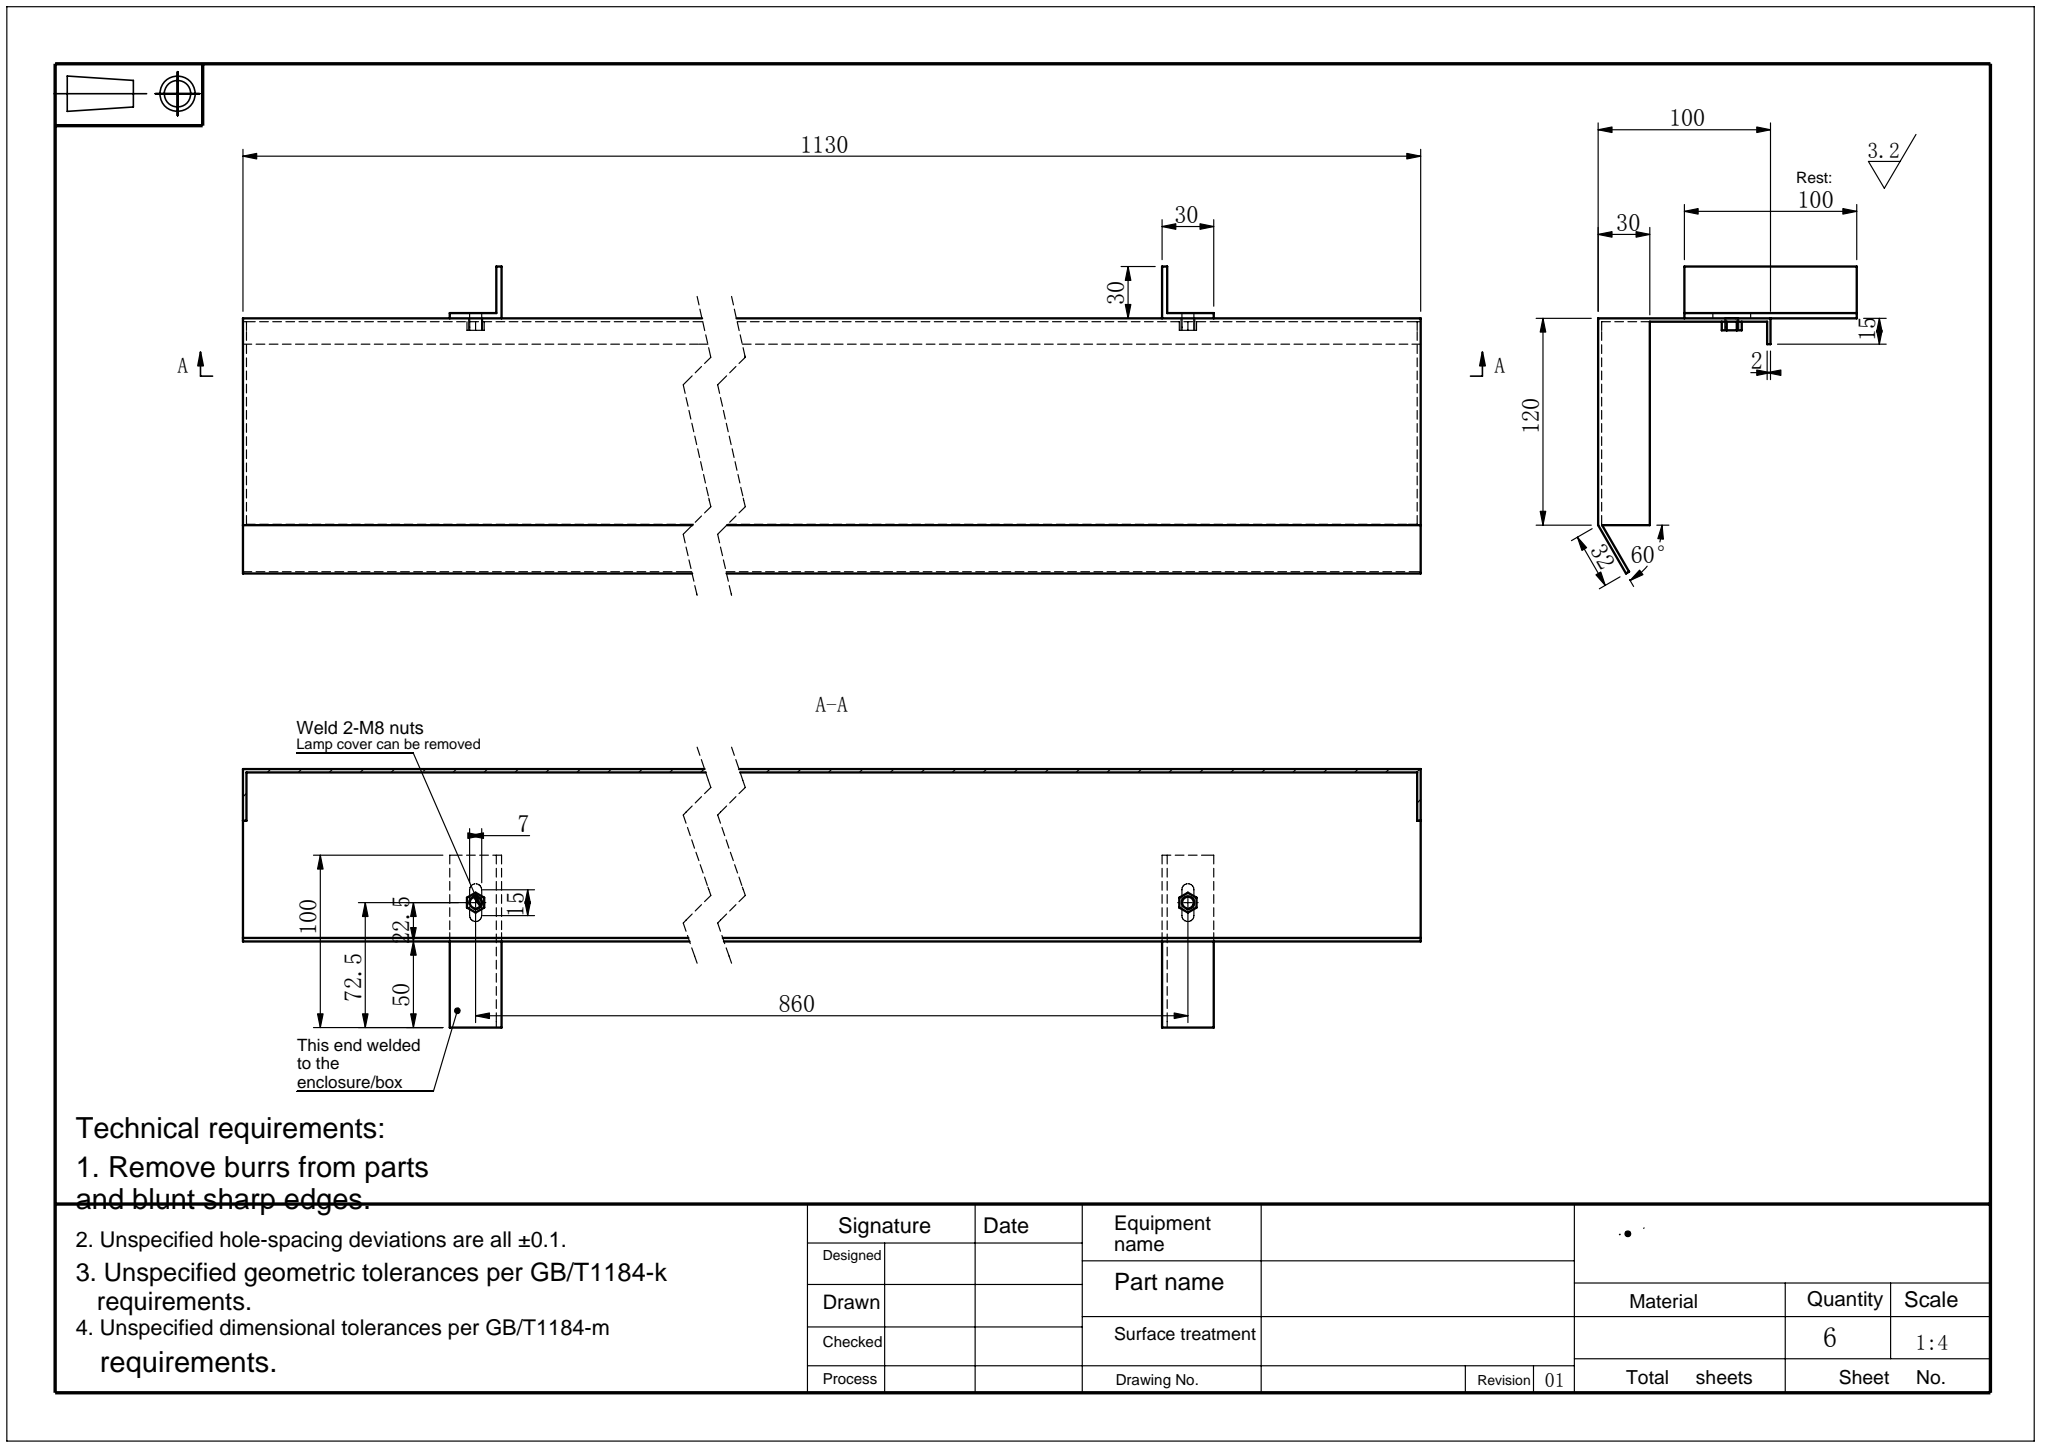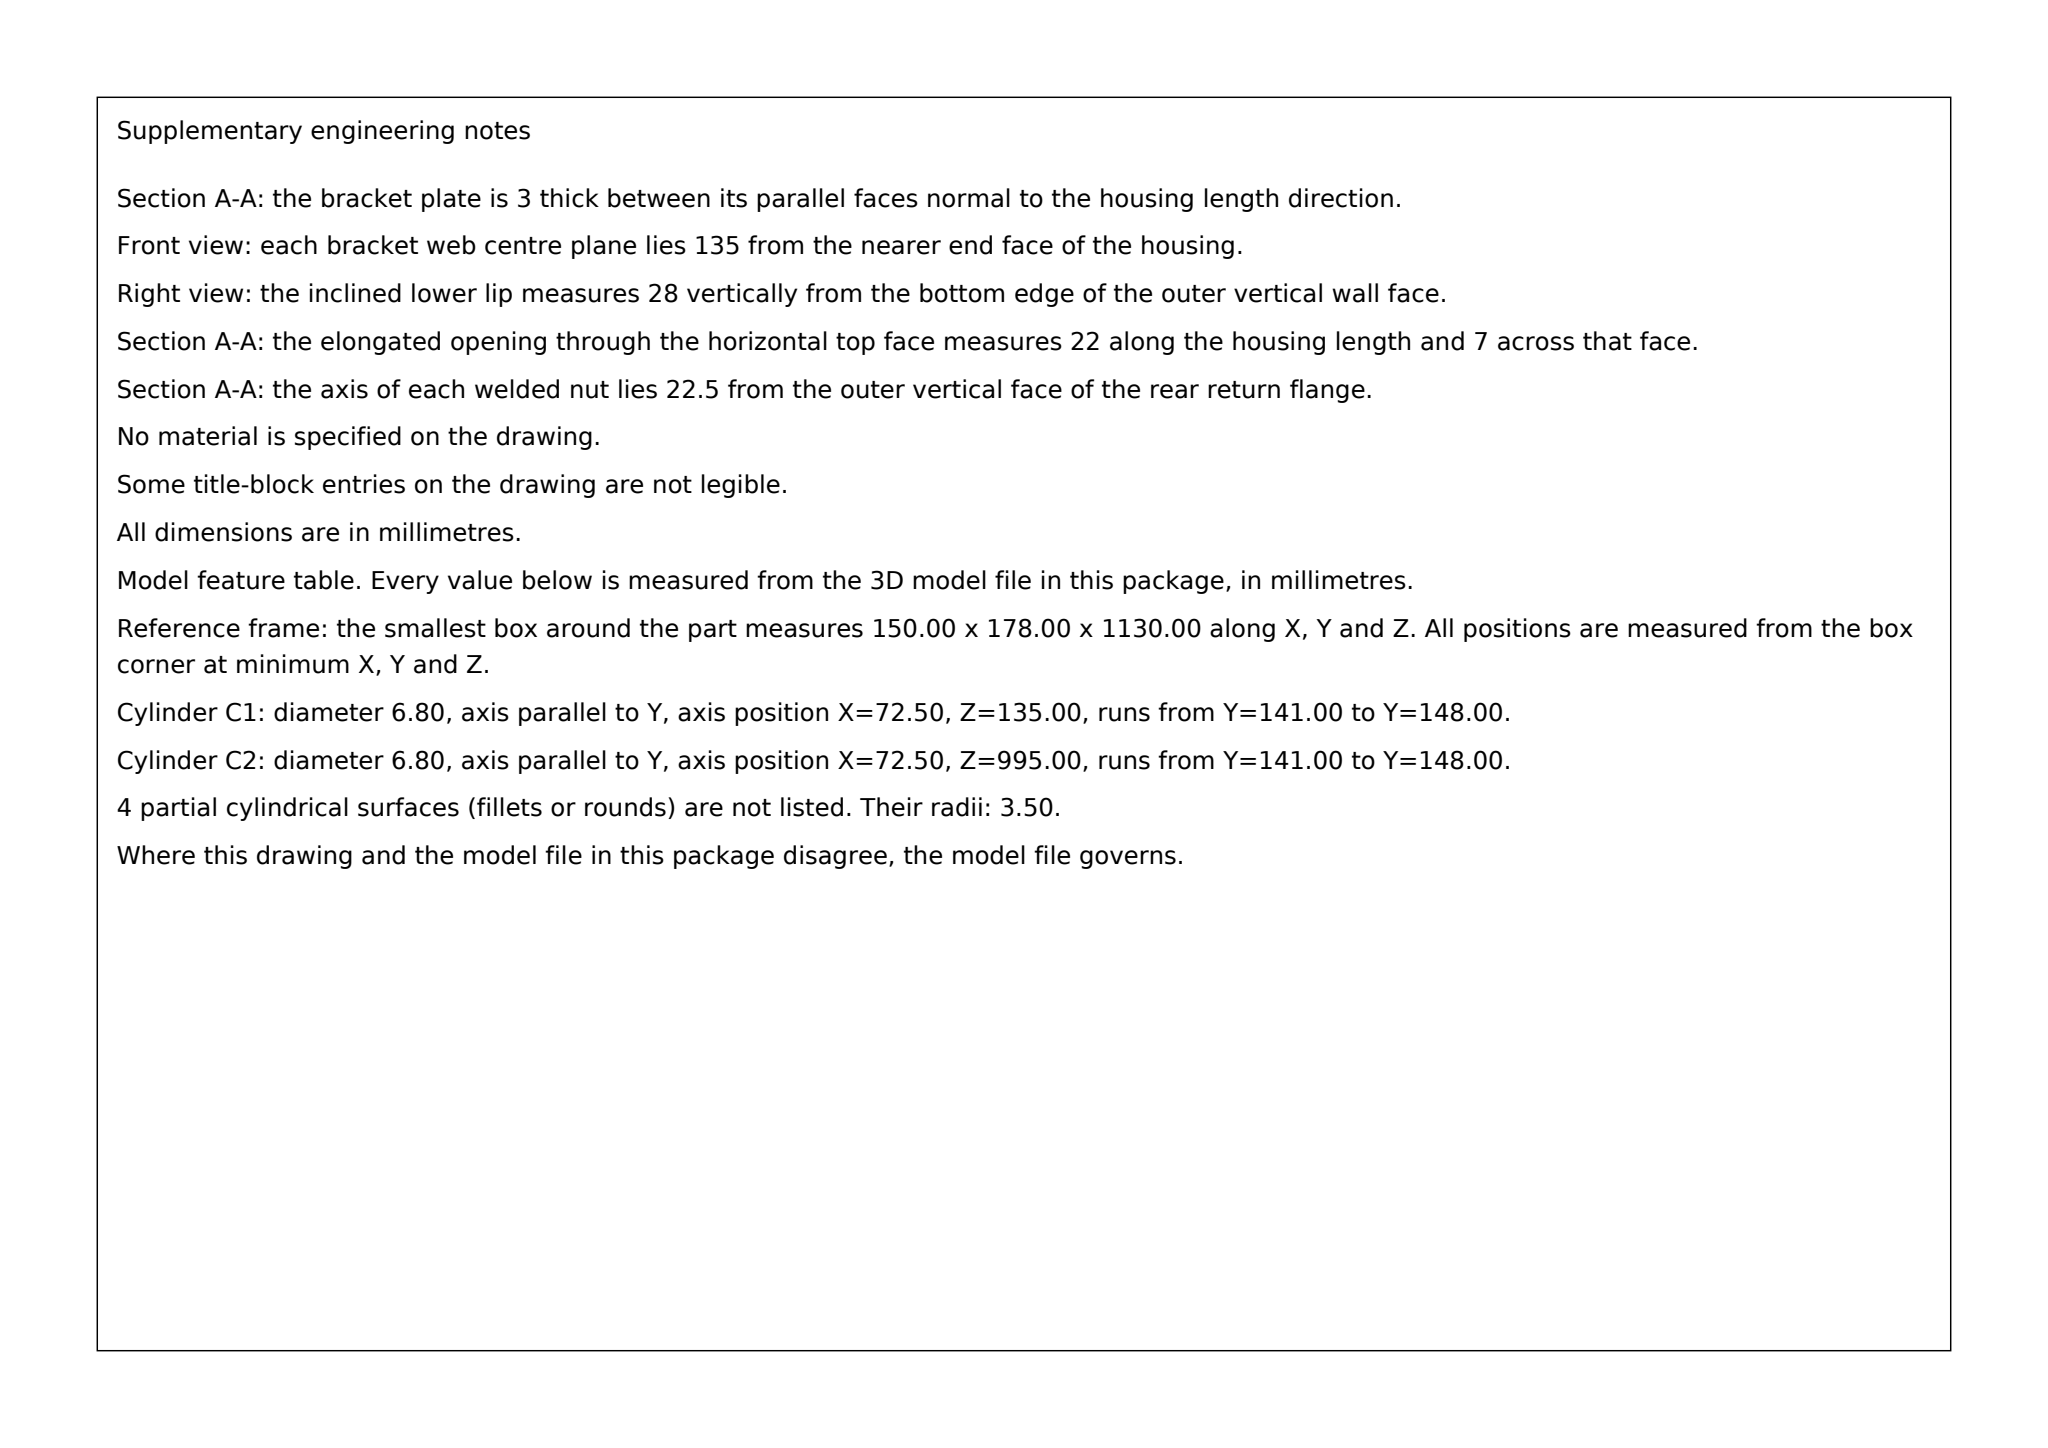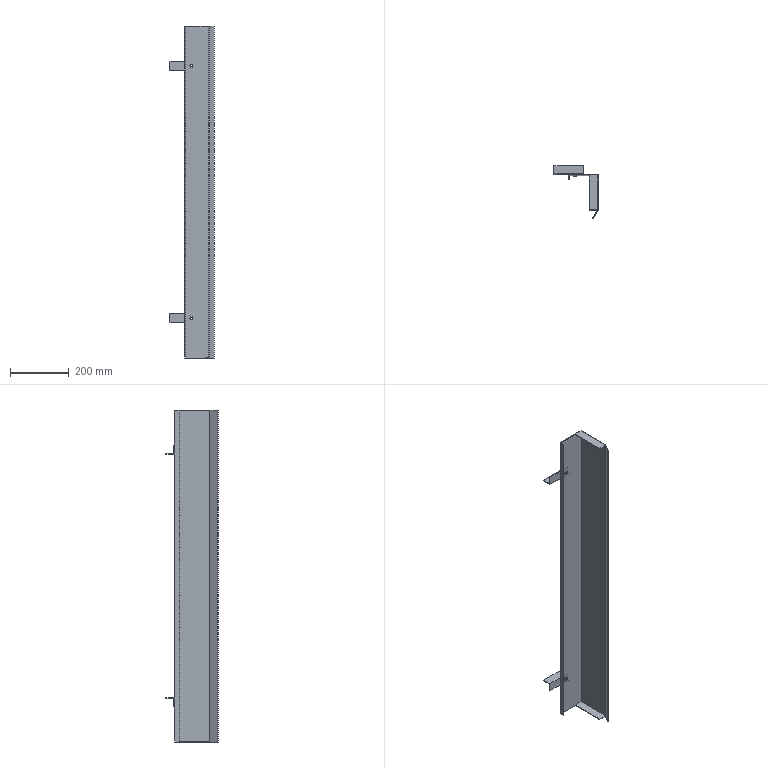Part | SolidWorks | mm | 1 solid | 62 faces | box 150 x 178 x 1130 mm | volume 640831 mm3 | plane 54 | cylinder 8 | commonest cylinder face diameters 6.8 x4 7 x4
build123d program:
from build123d import *

# Parameters (mm, degrees)
BOSS_EXTRUDE1_DEPTH = 565
SKETCH2_W           = 30
SKETCH2_H           = 120
BOSS_EXTRUDE2_DEPTH = 2
SKETCH3_W           = 30
SKETCH3_H           = 120
BOSS_EXTRUDE3_DEPTH = 2
BOSS_EXTRUDE5_DEPTH = 50
CUT_EXTRUDE3_DEPTH  = 3
BOSS_EXTRUDE6_DEPTH = 5


with BuildPart() as part:
    # Sketch1 → Boss-Extrude1 (new, symmetric)
    with BuildSketch(Plane.XY):
        Polygon((-20.263, 72.722), (-20.263, 87.722), (79.737, 87.722), (79.737, -32.278), (63.571, -60.278), (61.839, -59.278), (77.737, -31.742), (77.737, 85.722), (-18.263, 85.722), (-18.263, 72.722), align=None)
    extrude(amount=BOSS_EXTRUDE1_DEPTH, both=True)

    # Sketch2 → Boss-Extrude2 (add)
    with BuildSketch(Plane.XY.offset(565)):
        with Locations((64.737, 27.722)):
            Rectangle(SKETCH2_W, SKETCH2_H)
    extrude(amount=-BOSS_EXTRUDE2_DEPTH)

    # Sketch3 → Boss-Extrude3 (add)
    with BuildSketch(Plane(origin=(0, 0, -565), x_dir=(-1, 0, 0), z_dir=(0, 0, -1))):
        with Locations((-64.737, 27.722)):
            Rectangle(SKETCH3_W, SKETCH3_H)
    extrude(amount=-BOSS_EXTRUDE3_DEPTH)

    # Sketch8 → Boss-Extrude5 (add, symmetric)
    with BuildSketch(Plane.ZY.offset(20.263)):
        Polygon((415, 87.722), (415, 117.722), (418, 117.722), (418, 90.722), (445, 90.722), (445, 87.722), align=None)
    boss_extrude5 = extrude(amount=BOSS_EXTRUDE5_DEPTH, both=True)

    # Sketch9 → Cut-Extrude3 (cut)
    with BuildSketch(Plane(origin=(0, 90.722, 0), x_dir=(1, 0, 0), z_dir=(0, 1, 0))):
        with BuildLine():
            Line((-5.263, -426.5), (9.737, -426.5))
            ThreePointArc((9.737, -426.5), (13.237, -430), (9.737, -433.5))
            Line((9.737, -433.5), (-5.263, -433.5))
            ThreePointArc((-5.263, -433.5), (-8.763, -430), (-5.263, -426.5))
        make_face()
    cut_extrude3 = extrude(amount=-CUT_EXTRUDE3_DEPTH, mode=Mode.SUBTRACT)

    # Sketch11 → Boss-Extrude6 (add)
    with BuildSketch(Plane.XZ.offset(-85.722)):
        Polygon((8.01, 430), (5.123, 435), (-0.65, 435), (-3.537, 430), (-0.65, 425), (5.123, 425), align=None)
    boss_extrude6 = extrude(amount=BOSS_EXTRUDE6_DEPTH)

    # Sketch12 → M8 Tapped Hole1 (revolve, cut)
    with BuildSketch(Plane(origin=(2.237, 80.722, 430), x_dir=(0, 0, -1), z_dir=(1, 0, 0))):
        Polygon((0, 0), (0, 24.293), (3.4, 22.25), (3.4, 0), align=None)
    m8_tapped_hole1 = revolve(axis=Axis((2.237, 74.372, 430), (0, 1, 0)), mode=Mode.SUBTRACT)

    # Mirror3: Boss-Extrude5, Cut-Extrude3, Boss-Extrude6, M8 Tapped Hole1 across plane
    add(boss_extrude5.mirror(Plane.XY))
    add(cut_extrude3.mirror(Plane.XY), mode=Mode.SUBTRACT)
    add(boss_extrude6.mirror(Plane.XY))
    add(m8_tapped_hole1.mirror(Plane.XY), mode=Mode.SUBTRACT)


solid = part.part